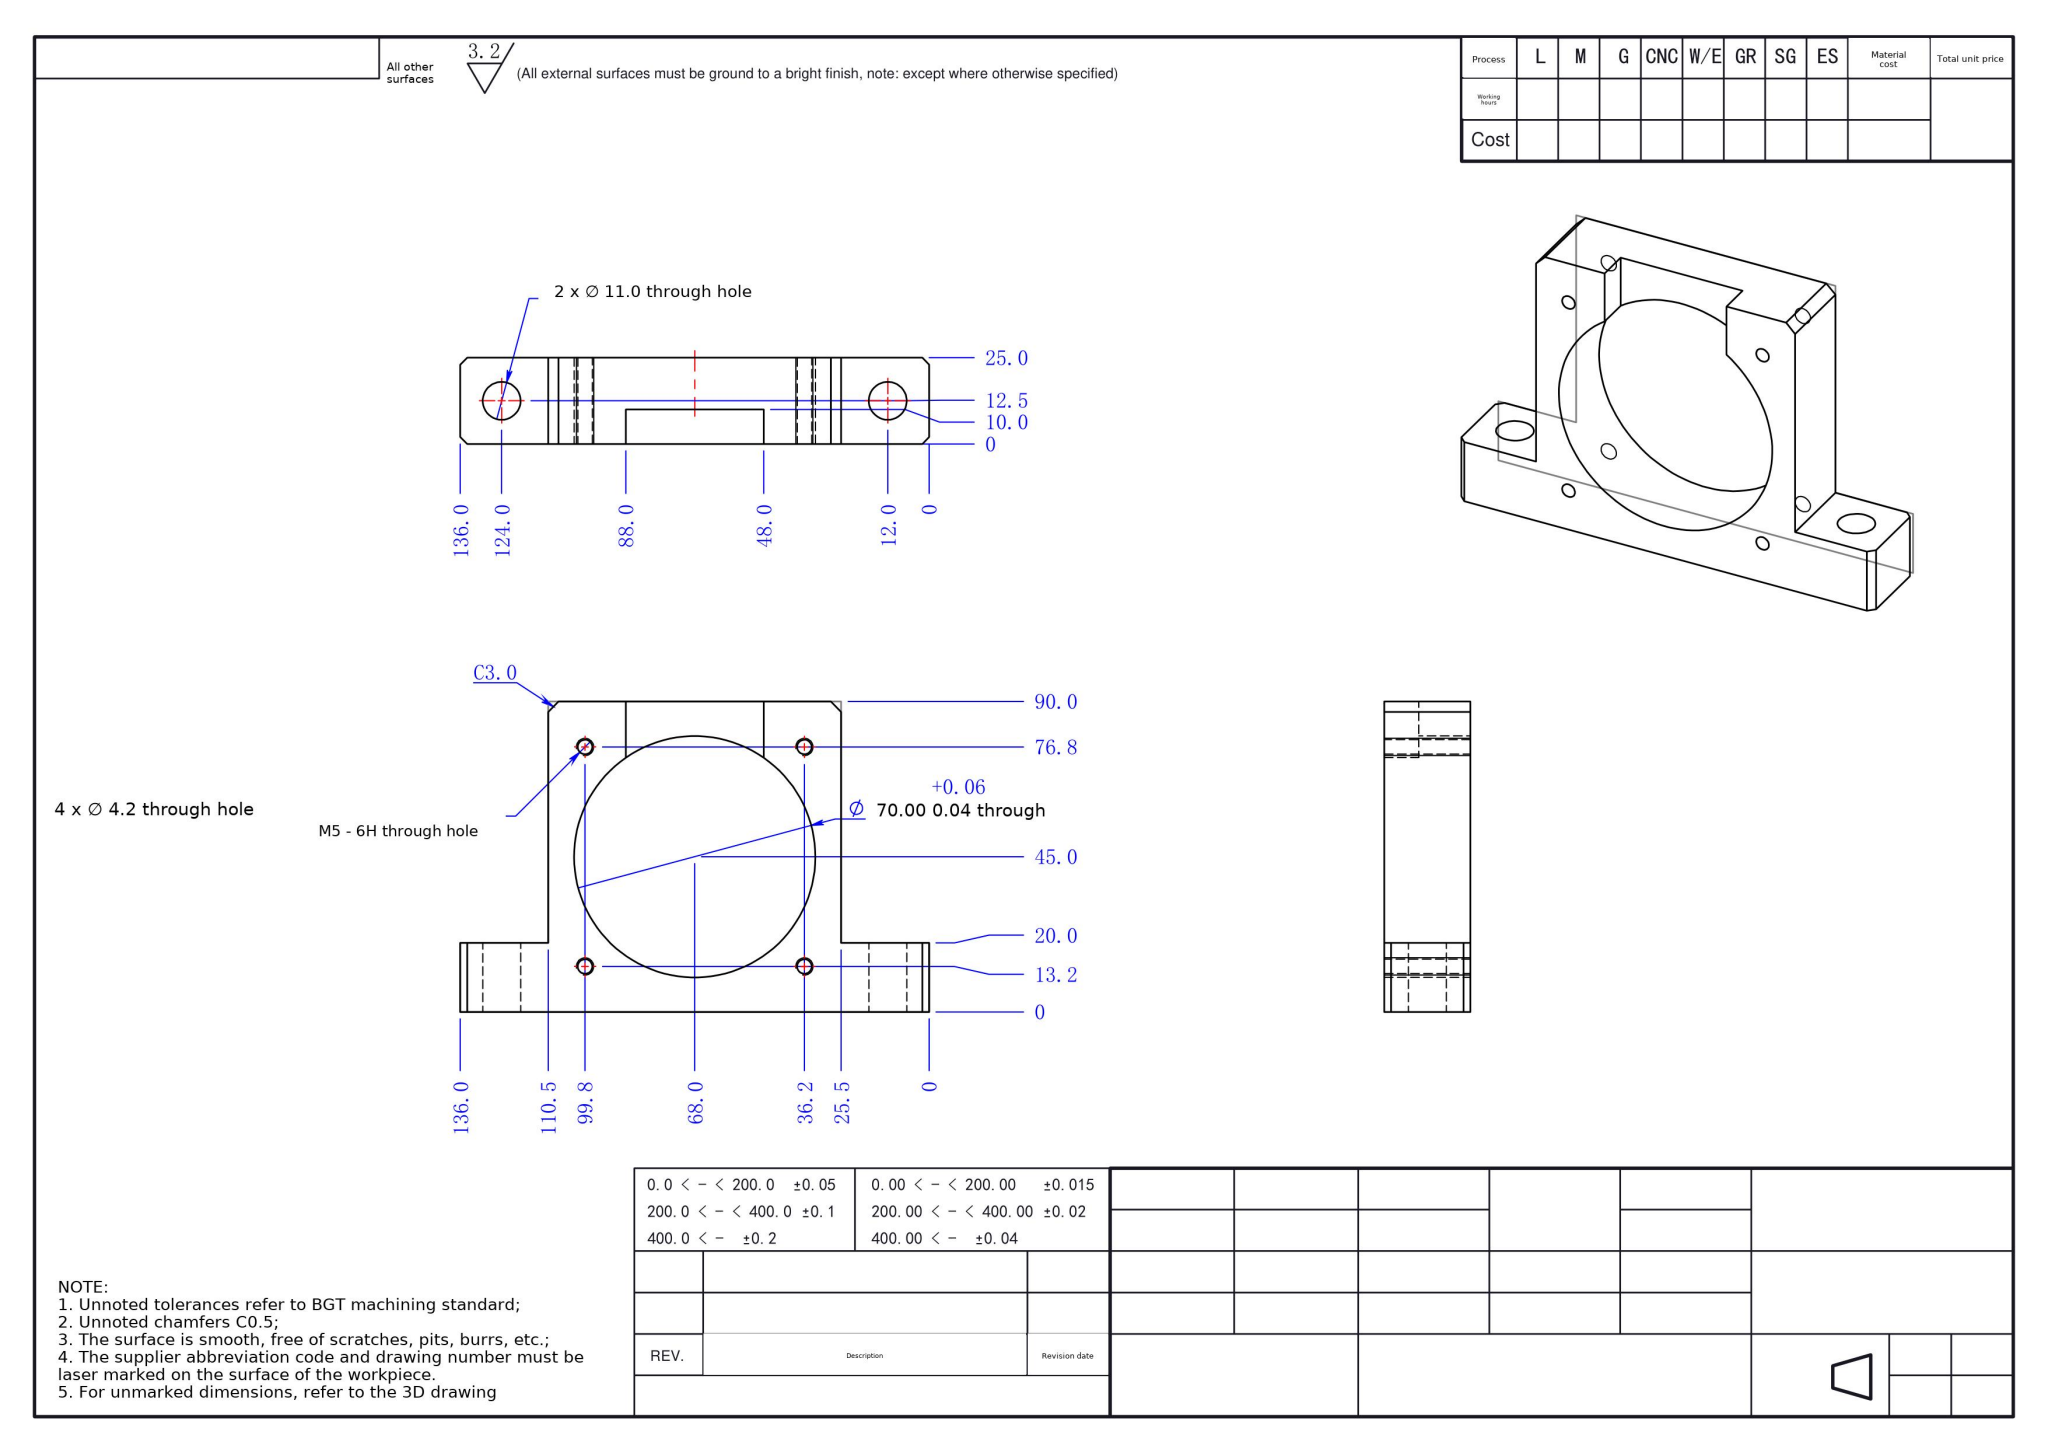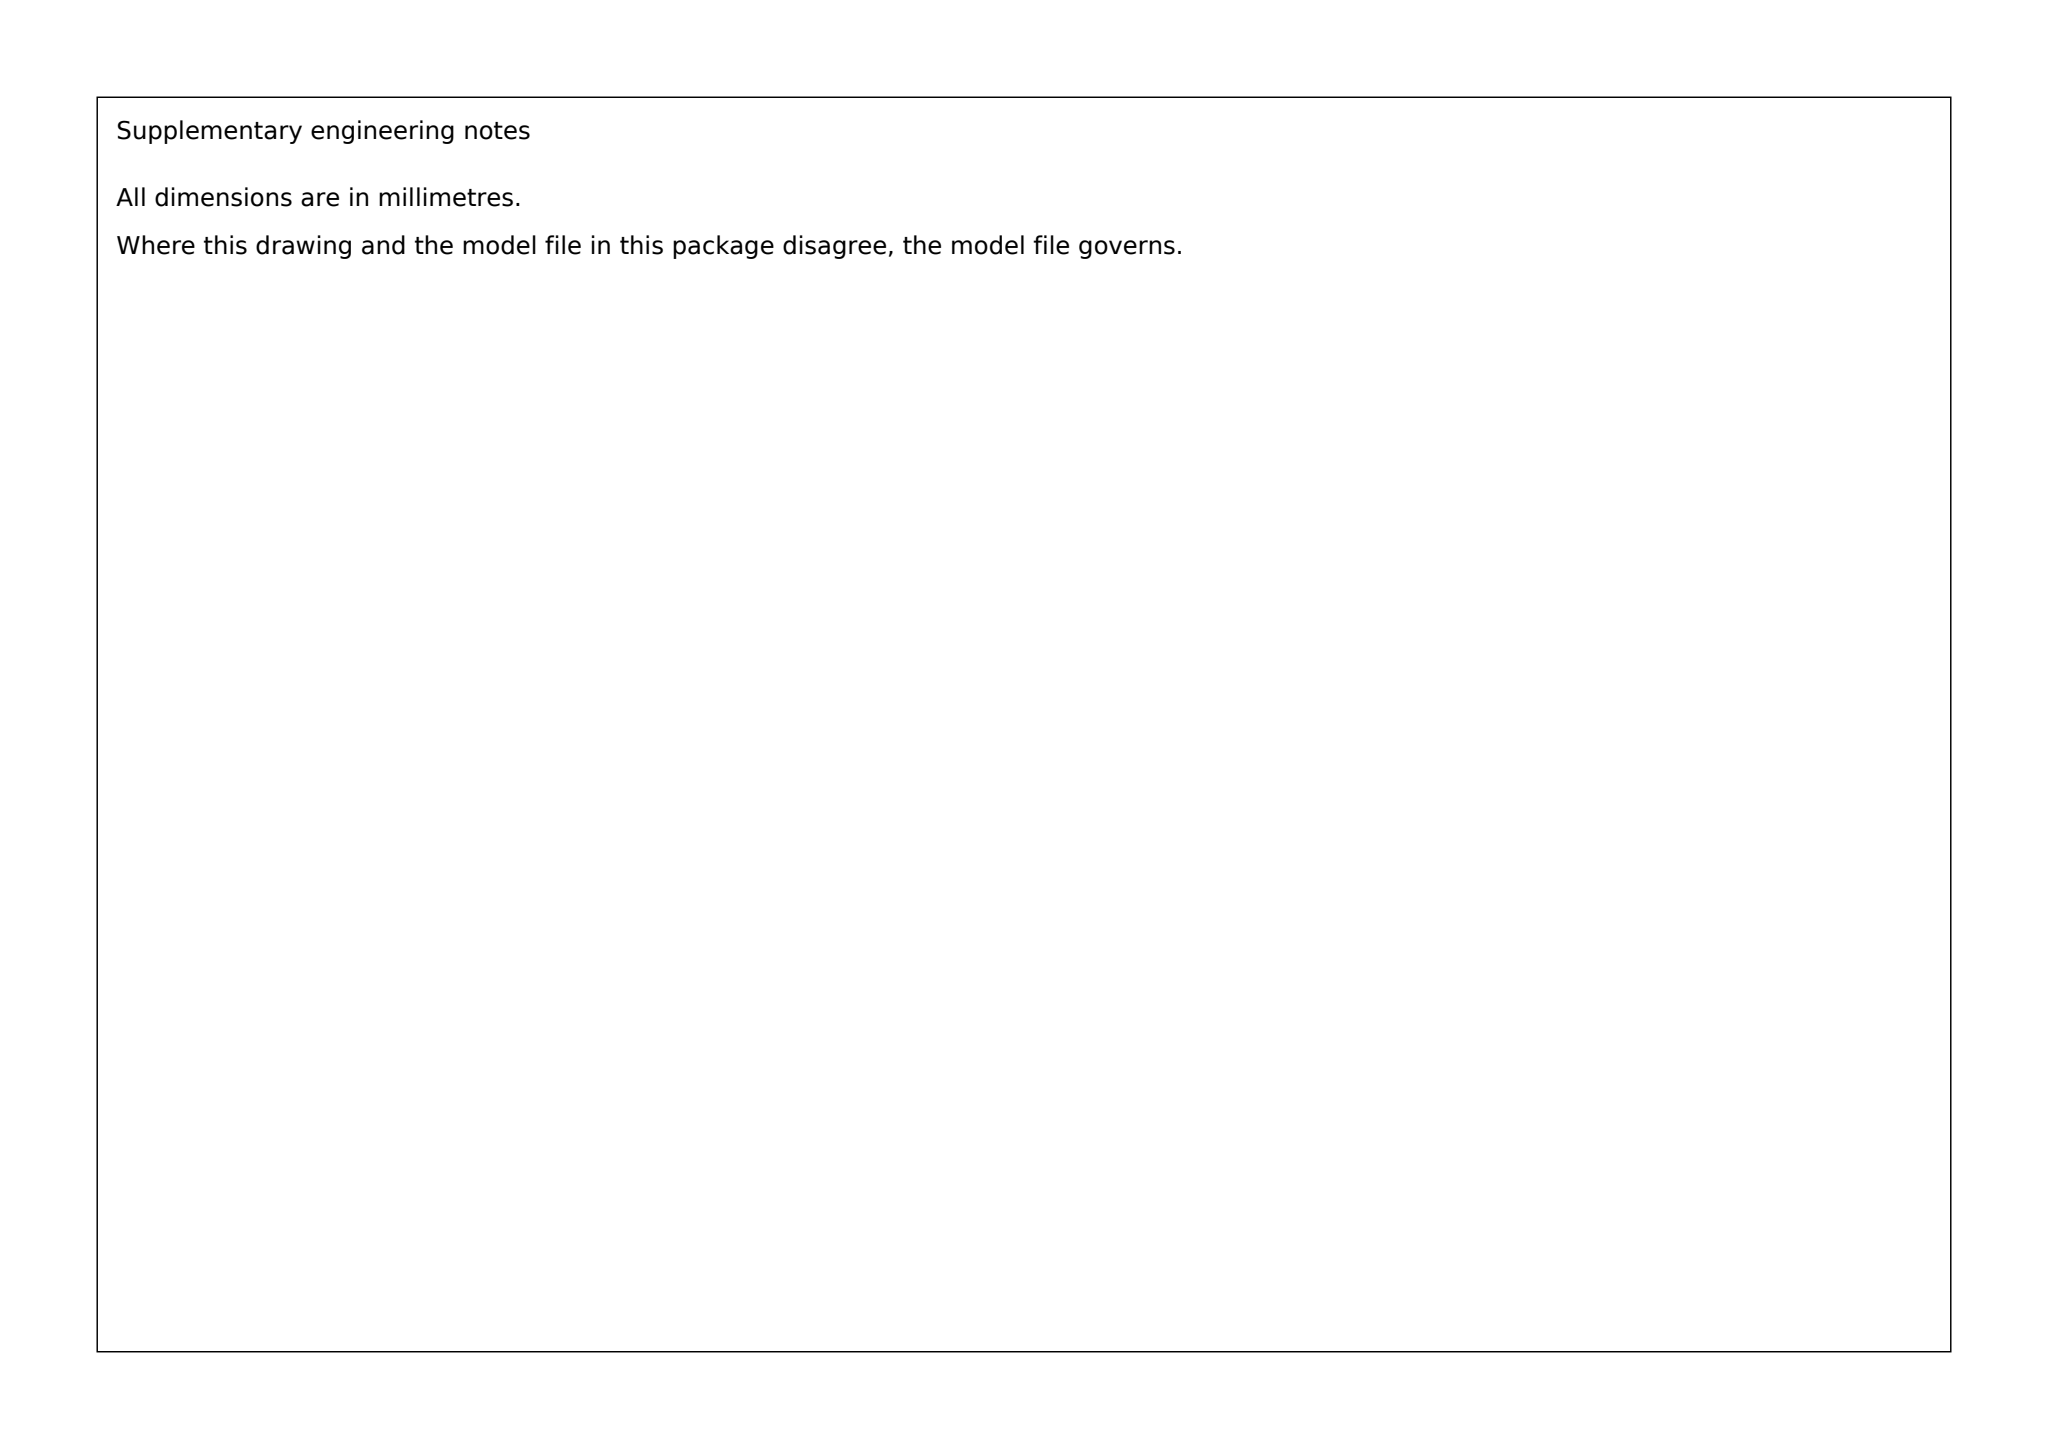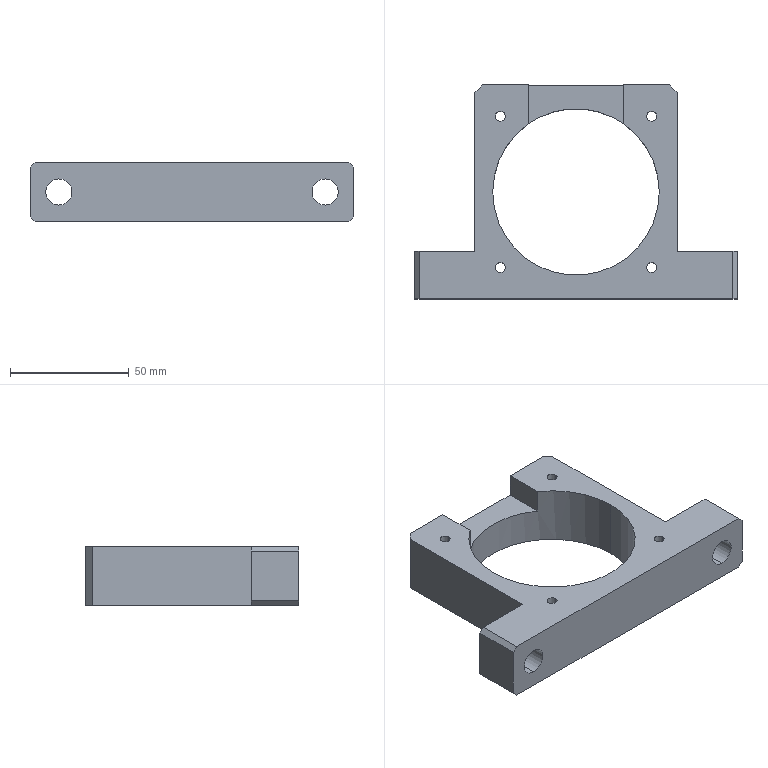Part | SolidWorks | mm | 1 solid | 33 faces | box 136 x 90 x 25 mm | volume 110163 mm3 | plane 19 | cylinder 14 | commonest cylinder face diameters 4.2 x8 11 x4 70 x2